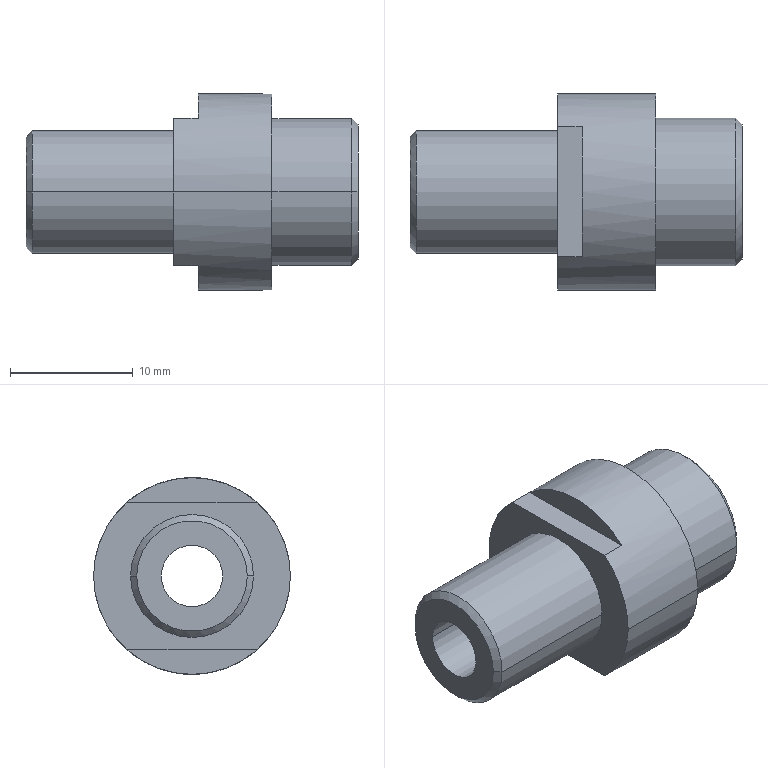Component | SolidWorks | ClampingAssembly-1_A72-1 | 1 solid | 20 faces | box 27 x 16 x 16 mm | volume 2746 mm3 | cylinder 8 | plane 8 | cone 4 | commonest cylinder face diameters 5 x2 10 x2 16 x2 12 x2 | material S45C
build123d program:
from build123d import *
from build123d.topology import SkipClean

# Parameters (mm, degrees)
SKETCH1_R             = 6
BOSS_EXTRUDE1_DEPTH   = 7
SKETCH2_R             = 8
BOSS_EXTRUDE2_DEPTH   = 6
CHAMFER1_SIZE         = 0.5
BOSS_EXTRUDE3_DEPTH   = 2
SKETCH4_R             = 5
BOSS_EXTRUDE4_DEPTH   = 12
M5_TAPPED_HOLE1_D     = 5
M5_TAPPED_HOLE1_DEPTH = 12.4
M5_TAPPED_HOLE1_TIP   = 1.502
M6_TAPPED_HOLE2_D     = 5
M6_TAPPED_HOLE2_DEPTH = 15
M6_TAPPED_HOLE2_TIP   = 1.502
CHAMFER2_SIZE         = 0.5


with BuildPart() as part:
    # Sketch1 → Boss-Extrude1 (new body)
    with BuildSketch(Plane(origin=(0, 0, 0), x_dir=(0, 0, -1), z_dir=(1, 0, 0))):
        Circle(SKETCH1_R)
    extrude(amount=BOSS_EXTRUDE1_DEPTH)

    # Sketch2 → Boss-Extrude2 (add)
    with BuildSketch(Plane.ZY):
        Circle(SKETCH2_R)
    extrude(amount=BOSS_EXTRUDE2_DEPTH)

    # Chamfer1
    chamfer1_edges = [part.edges().sort_by_distance(p)[0] for p in [
        (7, 0, 6),
    ]]
    chamfer(chamfer1_edges, length=CHAMFER1_SIZE)

    # Sketch3 → Boss-Extrude3 (add)
    with SkipClean():  # the faces are left unmerged after this step: merging them gives an invalid solid
        with BuildSketch(Plane.ZY.offset(6)):
            with BuildLine():
                Line((-5.292, 6), (5.292, 6))
                ThreePointArc((5.292, 6), (8, 0), (5.292, -6))
                Line((5.292, -6), (-5.292, -6))
                ThreePointArc((-5.292, -6), (-8, 0), (-5.292, 6))
            make_face()
        extrude(amount=BOSS_EXTRUDE3_DEPTH)

    # Sketch4 → Boss-Extrude4 (add)
    with SkipClean():  # the faces are left unmerged after this step: merging them gives an invalid solid
        with BuildSketch(Plane.ZY.offset(8)):
            Circle(SKETCH4_R)
        extrude(amount=BOSS_EXTRUDE4_DEPTH)

    # M5 Tapped Hole1
    with Locations(Plane(origin=(7, 0, 0), x_dir=(0, 0, -1), z_dir=(1, 0, 0))):
        with Locations((0, 0)):
            Hole(M5_TAPPED_HOLE1_D / 2, depth=M5_TAPPED_HOLE1_DEPTH)
            with Locations((0, 0, -(M5_TAPPED_HOLE1_DEPTH + M5_TAPPED_HOLE1_TIP / 2))):  # 118° drill point
                Cone(0, M5_TAPPED_HOLE1_D / 2, M5_TAPPED_HOLE1_TIP, mode=Mode.SUBTRACT)

    # M6 Tapped Hole2
    with Locations(Plane.ZY.offset(20)):
        with Locations((0, 0)):
            Hole(M6_TAPPED_HOLE2_D / 2, depth=M6_TAPPED_HOLE2_DEPTH)
            with Locations((0, 0, -(M6_TAPPED_HOLE2_DEPTH + M6_TAPPED_HOLE2_TIP / 2))):  # 118° drill point
                Cone(0, M6_TAPPED_HOLE2_D / 2, M6_TAPPED_HOLE2_TIP, mode=Mode.SUBTRACT)

    # Chamfer2
    chamfer2_edges = [part.edges().sort_by_distance(p)[0] for p in [
        (-20, 0, -5),
    ]]
    chamfer(chamfer2_edges, length=CHAMFER2_SIZE)


solid = part.part

# Placed as in the assembly
solid = solid.moved(Location((-29.551, 66.036, -52.5), (90, 0, 0)))
STEP:
#1=CARTESIAN_POINT('',(-1.951,2.777,-2.067));
#2=VERTEX_POINT('',#1);
#3=CARTESIAN_POINT('',(-1.951,2.423,-2.067));
#4=VERTEX_POINT('',#3);
#5=CARTESIAN_POINT('',(-1.951,2.6,-2.067));
#6=DIRECTION('',(-1.,-0.,-0.));
#7=DIRECTION('',(0.,1.,-0.0003333));
#8=AXIS2_PLACEMENT_3D('',#5,#6,#7);
#9=CIRCLE('',#8,0.1772);
#10=EDGE_CURVE('',#2,#4,#9,.T.);
#11=ORIENTED_EDGE('',*,*,#10,.F.);
#12=CARTESIAN_POINT('',(-1.931,2.797,-2.067));
#13=VERTEX_POINT('',#12);
#14=CARTESIAN_POINT('',(-1.951,2.777,-2.067));
#15=DIRECTION('',(0.7071,0.7071,-0.0002357));
#16=VECTOR('',#15,39.37);
#17=LINE('',#14,#16);
#18=EDGE_CURVE('',#2,#13,#17,.T.);
#19=ORIENTED_EDGE('',*,*,#18,.T.);
#20=CARTESIAN_POINT('',(-1.931,2.403,-2.067));
#21=VERTEX_POINT('',#20);
#22=CARTESIAN_POINT('',(-1.931,2.6,-2.067));
#23=DIRECTION('',(1.,0.,0.));
#24=DIRECTION('',(0.,1.,-0.0003333));
#25=AXIS2_PLACEMENT_3D('',#22,#23,#24);
#26=CIRCLE('',#25,0.1969);
#27=EDGE_CURVE('',#21,#13,#26,.T.);
#28=ORIENTED_EDGE('',*,*,#27,.F.);
#29=CARTESIAN_POINT('',(-1.951,2.423,-2.067));
#30=DIRECTION('',(0.7071,-0.7071,0.0002357));
#31=VECTOR('',#30,39.37);
#32=LINE('',#29,#31);
#33=EDGE_CURVE('',#4,#21,#32,.T.);
#34=ORIENTED_EDGE('',*,*,#33,.F.);
#35=EDGE_LOOP('',(#11,#19,#28,#34));
#36=FACE_OUTER_BOUND('',#35,.T.);
#37=CARTESIAN_POINT('',(-1.951,2.6,-2.067));
#38=DIRECTION('',(1.,0.,0.));
#39=DIRECTION('',(0.,-1.,0.0003333));
#40=AXIS2_PLACEMENT_3D('',#37,#38,#39);
#41=CONICAL_SURFACE('',#40,0.1772,0.7854);
#42=ADVANCED_FACE('',(#36),#41,.T.);
#43=CARTESIAN_POINT('',(-1.951,2.501,-2.067));
#44=VERTEX_POINT('',#43);
#45=CARTESIAN_POINT('',(-1.951,2.698,-2.067));
#46=VERTEX_POINT('',#45);
#47=CARTESIAN_POINT('',(-1.951,2.6,-2.067));
#48=DIRECTION('',(-1.,-0.,-0.));
#49=DIRECTION('',(0.,1.,-0.0003333));
#50=AXIS2_PLACEMENT_3D('',#47,#48,#49);
#51=CIRCLE('',#50,0.09843);
#52=EDGE_CURVE('',#44,#46,#51,.T.);
#53=ORIENTED_EDGE('',*,*,#52,.T.);
#54=CARTESIAN_POINT('',(-0.8878,2.698,-2.067));
#55=VERTEX_POINT('',#54);
#56=CARTESIAN_POINT('',(-0.8878,2.698,-2.067));
#57=DIRECTION('',(1.,0.,0.));
#58=VECTOR('',#57,39.37);
#59=LINE('',#56,#58);
#60=EDGE_CURVE('',#46,#55,#59,.T.);
#61=ORIENTED_EDGE('',*,*,#60,.T.);
#62=CARTESIAN_POINT('',(-0.8878,2.501,-2.067));
#63=VERTEX_POINT('',#62);
#64=CARTESIAN_POINT('',(-0.8878,2.6,-2.067));
#65=DIRECTION('',(1.,0.,0.));
#66=DIRECTION('',(0.,-1.,0.0003333));
#67=AXIS2_PLACEMENT_3D('',#64,#65,#66);
#68=CIRCLE('',#67,0.09843);
#69=EDGE_CURVE('',#55,#63,#68,.T.);
#70=ORIENTED_EDGE('',*,*,#69,.T.);
#71=CARTESIAN_POINT('',(-0.8878,2.501,-2.067));
#72=DIRECTION('',(1.,0.,0.));
#73=VECTOR('',#72,39.37);
#74=LINE('',#71,#73);
#75=EDGE_CURVE('',#44,#63,#74,.T.);
#76=ORIENTED_EDGE('',*,*,#75,.F.);
#77=EDGE_LOOP('',(#53,#61,#70,#76));
#78=FACE_OUTER_BOUND('',#77,.T.);
#79=CARTESIAN_POINT('',(-0.8878,2.6,-2.067));
#80=DIRECTION('',(1.,0.,0.));
#81=DIRECTION('',(0.,-1.,0.0003333));
#82=AXIS2_PLACEMENT_3D('',#79,#80,#81);
#83=CYLINDRICAL_SURFACE('',#82,0.09843);
#84=ADVANCED_FACE('',(#78),#83,.F.);
#85=ORIENTED_EDGE('',*,*,#27,.T.);
#86=CARTESIAN_POINT('',(-1.478,2.797,-2.067));
#87=VERTEX_POINT('',#86);
#88=CARTESIAN_POINT('',(-1.951,2.797,-2.067));
#89=DIRECTION('',(1.,0.,0.));
#90=VECTOR('',#89,39.37);
#91=LINE('',#88,#90);
#92=EDGE_CURVE('',#13,#87,#91,.T.);
#93=ORIENTED_EDGE('',*,*,#92,.T.);
#94=CARTESIAN_POINT('',(-1.478,2.403,-2.067));
#95=VERTEX_POINT('',#94);
#96=CARTESIAN_POINT('',(-1.478,2.6,-2.067));
#97=DIRECTION('',(-1.,-0.,-0.));
#98=DIRECTION('',(0.,1.,-0.0003333));
#99=AXIS2_PLACEMENT_3D('',#96,#97,#98);
#100=CIRCLE('',#99,0.1969);
#101=EDGE_CURVE('',#87,#95,#100,.T.);
#102=ORIENTED_EDGE('',*,*,#101,.T.);
#103=CARTESIAN_POINT('',(-1.951,2.403,-2.067));
#104=DIRECTION('',(1.,0.,0.));
#105=VECTOR('',#104,39.37);
#106=LINE('',#103,#105);
#107=EDGE_CURVE('',#21,#95,#106,.T.);
#108=ORIENTED_EDGE('',*,*,#107,.F.);
#109=EDGE_LOOP('',(#85,#93,#102,#108));
#110=FACE_OUTER_BOUND('',#109,.T.);
#111=CARTESIAN_POINT('',(-1.951,2.6,-2.067));
#112=DIRECTION('',(1.,0.,0.));
#113=DIRECTION('',(0.,-1.,0.0003333));
#114=AXIS2_PLACEMENT_3D('',#111,#112,#113);
#115=CYLINDRICAL_SURFACE('',#114,0.1969);
#116=ADVANCED_FACE('',(#110),#115,.T.);
#117=CARTESIAN_POINT('',(-0.8878,2.383,-2.067));
#118=VERTEX_POINT('',#117);
#119=CARTESIAN_POINT('',(-0.8878,2.816,-2.067));
#120=VERTEX_POINT('',#119);
#121=CARTESIAN_POINT('',(-0.8878,2.6,-2.067));
#122=DIRECTION('',(1.,0.,0.));
#123=DIRECTION('',(0.,-1.,0.0003333));
#124=AXIS2_PLACEMENT_3D('',#121,#122,#123);
#125=CIRCLE('',#124,0.2165);
#126=EDGE_CURVE('',#118,#120,#125,.T.);
#127=ORIENTED_EDGE('',*,*,#126,.F.);
#128=CARTESIAN_POINT('',(-0.9075,2.364,-2.067));
#129=VERTEX_POINT('',#128);
#130=CARTESIAN_POINT('',(-0.8878,2.383,-2.067));
#131=DIRECTION('',(-0.7071,-0.7071,0.0002357));
#132=VECTOR('',#131,39.37);
#133=LINE('',#130,#132);
#134=EDGE_CURVE('',#118,#129,#133,.T.);
#135=ORIENTED_EDGE('',*,*,#134,.T.);
#136=CARTESIAN_POINT('',(-0.9075,2.836,-2.067));
#137=VERTEX_POINT('',#136);
#138=CARTESIAN_POINT('',(-0.9075,2.6,-2.067));
#139=DIRECTION('',(-1.,-0.,-0.));
#140=DIRECTION('',(0.,-1.,0.0003333));
#141=AXIS2_PLACEMENT_3D('',#138,#139,#140);
#142=CIRCLE('',#141,0.2362);
#143=EDGE_CURVE('',#137,#129,#142,.T.);
#144=ORIENTED_EDGE('',*,*,#143,.F.);
#145=CARTESIAN_POINT('',(-0.8878,2.816,-2.067));
#146=DIRECTION('',(-0.7071,0.7071,-0.0002357));
#147=VECTOR('',#146,39.37);
#148=LINE('',#145,#147);
#149=EDGE_CURVE('',#120,#137,#148,.T.);
#150=ORIENTED_EDGE('',*,*,#149,.F.);
#151=EDGE_LOOP('',(#127,#135,#144,#150));
#152=FACE_OUTER_BOUND('',#151,.T.);
#153=CARTESIAN_POINT('',(-0.8878,2.6,-2.067));
#154=DIRECTION('',(-1.,-0.,-0.));
#155=DIRECTION('',(0.,1.,-0.0003333));
#156=AXIS2_PLACEMENT_3D('',#153,#154,#155);
#157=CONICAL_SURFACE('',#156,0.2165,0.7854);
#158=ADVANCED_FACE('',(#152),#157,.T.);
#159=CARTESIAN_POINT('',(-1.478,2.915,-2.067));
#160=VERTEX_POINT('',#159);
#161=CARTESIAN_POINT('',(-1.478,2.808,-2.303));
#162=VERTEX_POINT('',#161);
#163=CARTESIAN_POINT('',(-1.478,2.6,-2.067));
#164=DIRECTION('',(-1.,-0.,-0.));
#165=DIRECTION('',(0.,1.,-0.0003333));
#166=AXIS2_PLACEMENT_3D('',#163,#164,#165);
#167=CIRCLE('',#166,0.315);
#168=EDGE_CURVE('',#160,#162,#167,.T.);
#169=ORIENTED_EDGE('',*,*,#168,.F.);
#170=CARTESIAN_POINT('',(-1.163,2.915,-2.067));
#171=VERTEX_POINT('',#170);
#172=CARTESIAN_POINT('',(-1.4,2.915,-2.067));
#173=DIRECTION('',(1.,0.,0.));
#174=VECTOR('',#173,39.37);
#175=LINE('',#172,#174);
#176=EDGE_CURVE('',#160,#171,#175,.T.);
#177=ORIENTED_EDGE('',*,*,#176,.T.);
#178=CARTESIAN_POINT('',(-1.163,2.285,-2.067));
#179=VERTEX_POINT('',#178);
#180=CARTESIAN_POINT('',(-1.163,2.6,-2.067));
#181=DIRECTION('',(-1.,-0.,-0.));
#182=DIRECTION('',(0.,1.,-0.0003333));
#183=AXIS2_PLACEMENT_3D('',#180,#181,#182);
#184=CIRCLE('',#183,0.315);
#185=EDGE_CURVE('',#171,#179,#184,.T.);
#186=ORIENTED_EDGE('',*,*,#185,.T.);
#187=CARTESIAN_POINT('',(-1.478,2.285,-2.067));
#188=VERTEX_POINT('',#187);
#189=CARTESIAN_POINT('',(-1.4,2.285,-2.067));
#190=DIRECTION('',(1.,0.,0.));
#191=VECTOR('',#190,39.37);
#192=LINE('',#189,#191);
#193=EDGE_CURVE('',#188,#179,#192,.T.);
#194=ORIENTED_EDGE('',*,*,#193,.F.);
#195=CARTESIAN_POINT('',(-1.478,2.391,-2.303));
#196=VERTEX_POINT('',#195);
#197=CARTESIAN_POINT('',(-1.478,2.6,-2.067));
#198=DIRECTION('',(-1.,-0.,-0.));
#199=DIRECTION('',(0.,1.,-0.0003333));
#200=AXIS2_PLACEMENT_3D('',#197,#198,#199);
#201=CIRCLE('',#200,0.315);
#202=EDGE_CURVE('',#196,#188,#201,.T.);
#203=ORIENTED_EDGE('',*,*,#202,.F.);
#204=CARTESIAN_POINT('',(-1.4,2.391,-2.303));
#205=VERTEX_POINT('',#204);
#206=CARTESIAN_POINT('',(-1.478,2.391,-2.303));
#207=DIRECTION('',(1.,0.,0.));
#208=VECTOR('',#207,39.37);
#209=LINE('',#206,#208);
#210=EDGE_CURVE('',#196,#205,#209,.T.);
#211=ORIENTED_EDGE('',*,*,#210,.T.);
#212=CARTESIAN_POINT('',(-1.4,2.808,-2.303));
#213=VERTEX_POINT('',#212);
#214=CARTESIAN_POINT('',(-1.4,2.6,-2.067));
#215=DIRECTION('',(-1.,-0.,-0.));
#216=DIRECTION('',(0.,1.,-0.0003333));
#217=AXIS2_PLACEMENT_3D('',#214,#215,#216);
#218=CIRCLE('',#217,0.315);
#219=EDGE_CURVE('',#213,#205,#218,.T.);
#220=ORIENTED_EDGE('',*,*,#219,.F.);
#221=CARTESIAN_POINT('',(-1.478,2.808,-2.303));
#222=DIRECTION('',(1.,0.,0.));
#223=VECTOR('',#222,39.37);
#224=LINE('',#221,#223);
#225=EDGE_CURVE('',#162,#213,#224,.T.);
#226=ORIENTED_EDGE('',*,*,#225,.F.);
#227=EDGE_LOOP('',(#169,#177,#186,#194,#203,#211,#220,#226));
#228=FACE_OUTER_BOUND('',#227,.T.);
#229=CARTESIAN_POINT('',(-1.4,2.6,-2.067));
#230=DIRECTION('',(1.,0.,0.));
#231=DIRECTION('',(0.,-1.,0.0003333));
#232=AXIS2_PLACEMENT_3D('',#229,#230,#231);
#233=CYLINDRICAL_SURFACE('',#232,0.315);
#234=ADVANCED_FACE('',(#228),#233,.T.);
#235=ORIENTED_EDGE('',*,*,#143,.T.);
#236=CARTESIAN_POINT('',(-1.163,2.364,-2.067));
#237=VERTEX_POINT('',#236);
#238=CARTESIAN_POINT('',(-0.8878,2.364,-2.067));
#239=DIRECTION('',(-1.,-0.,-0.));
#240=VECTOR('',#239,39.37);
#241=LINE('',#238,#240);
#242=EDGE_CURVE('',#129,#237,#241,.T.);
#243=ORIENTED_EDGE('',*,*,#242,.T.);
#244=CARTESIAN_POINT('',(-1.163,2.836,-2.067));
#245=VERTEX_POINT('',#244);
#246=CARTESIAN_POINT('',(-1.163,2.6,-2.067));
#247=DIRECTION('',(1.,0.,0.));
#248=DIRECTION('',(0.,-1.,0.0003333));
#249=AXIS2_PLACEMENT_3D('',#246,#247,#248);
#250=CIRCLE('',#249,0.2362);
#251=EDGE_CURVE('',#237,#245,#250,.T.);
#252=ORIENTED_EDGE('',*,*,#251,.T.);
#253=CARTESIAN_POINT('',(-0.8878,2.836,-2.067));
#254=DIRECTION('',(-1.,-0.,-0.));
#255=VECTOR('',#254,39.37);
#256=LINE('',#253,#255);
#257=EDGE_CURVE('',#137,#245,#256,.T.);
#258=ORIENTED_EDGE('',*,*,#257,.F.);
#259=EDGE_LOOP('',(#235,#243,#252,#258));
#260=FACE_OUTER_BOUND('',#259,.T.);
#261=CARTESIAN_POINT('',(-0.8878,2.6,-2.067));
#262=DIRECTION('',(-1.,-0.,-0.));
#263=DIRECTION('',(0.,1.,-0.0003333));
#264=AXIS2_PLACEMENT_3D('',#261,#262,#263);
#265=CYLINDRICAL_SURFACE('',#264,0.2362);
#266=ADVANCED_FACE('',(#260),#265,.T.);
#267=CARTESIAN_POINT('',(-1.4,2.391,-2.303));
#268=DIRECTION('',(0.,-1.,0.0003333));
#269=VECTOR('',#268,39.37);
#270=LINE('',#267,#269);
#271=EDGE_CURVE('',#213,#205,#270,.T.);
#272=ORIENTED_EDGE('',*,*,#271,.F.);
#273=ORIENTED_EDGE('',*,*,#219,.T.);
#274=EDGE_LOOP('',(#272,#273));
#275=FACE_OUTER_BOUND('',#274,.T.);
#276=CARTESIAN_POINT('',(-1.4,2.6,-2.067));
#277=DIRECTION('',(-1.,-0.,-0.));
#278=DIRECTION('',(-0.,1.,-0.0003333));
#279=AXIS2_PLACEMENT_3D('',#276,#277,#278);
#280=PLANE('',#279);
#281=ADVANCED_FACE('',(#275),#280,.T.);
#282=ORIENTED_EDGE('',*,*,#242,.F.);
#283=CARTESIAN_POINT('',(-0.9075,2.6,-2.067));
#284=DIRECTION('',(-1.,-0.,-0.));
#285=DIRECTION('',(0.,-1.,0.0003333));
#286=AXIS2_PLACEMENT_3D('',#283,#284,#285);
#287=CIRCLE('',#286,0.2362);
#288=EDGE_CURVE('',#129,#137,#287,.T.);
#289=ORIENTED_EDGE('',*,*,#288,.T.);
#290=ORIENTED_EDGE('',*,*,#257,.T.);
#291=CARTESIAN_POINT('',(-1.163,2.6,-2.067));
#292=DIRECTION('',(1.,0.,0.));
#293=DIRECTION('',(0.,-1.,0.0003333));
#294=AXIS2_PLACEMENT_3D('',#291,#292,#293);
#295=CIRCLE('',#294,0.2362);
#296=EDGE_CURVE('',#245,#237,#295,.T.);
#297=ORIENTED_EDGE('',*,*,#296,.T.);
#298=EDGE_LOOP('',(#282,#289,#290,#297));
#299=FACE_OUTER_BOUND('',#298,.T.);
#300=CARTESIAN_POINT('',(-0.8878,2.6,-2.067));
#301=DIRECTION('',(-1.,-0.,-0.));
#302=DIRECTION('',(0.,1.,-0.0003333));
#303=AXIS2_PLACEMENT_3D('',#300,#301,#302);
#304=CYLINDRICAL_SURFACE('',#303,0.2362);
#305=ADVANCED_FACE('',(#299),#304,.T.);
#306=CARTESIAN_POINT('',(-0.8878,2.6,-2.067));
#307=DIRECTION('',(1.,0.,0.));
#308=DIRECTION('',(0.,-1.,0.0003333));
#309=AXIS2_PLACEMENT_3D('',#306,#307,#308);
#310=CIRCLE('',#309,0.09843);
#311=EDGE_CURVE('',#63,#55,#310,.T.);
#312=ORIENTED_EDGE('',*,*,#311,.F.);
#313=ORIENTED_EDGE('',*,*,#69,.F.);
#314=EDGE_LOOP('',(#312,#313));
#315=FACE_BOUND('',#314,.T.);
#316=CARTESIAN_POINT('',(-0.8878,2.6,-2.067));
#317=DIRECTION('',(1.,0.,0.));
#318=DIRECTION('',(0.,-1.,0.0003333));
#319=AXIS2_PLACEMENT_3D('',#316,#317,#318);
#320=CIRCLE('',#319,0.2165);
#321=EDGE_CURVE('',#120,#118,#320,.T.);
#322=ORIENTED_EDGE('',*,*,#321,.T.);
#323=ORIENTED_EDGE('',*,*,#126,.T.);
#324=EDGE_LOOP('',(#322,#323));
#325=FACE_OUTER_BOUND('',#324,.T.);
#326=CARTESIAN_POINT('',(-0.8878,2.6,-2.067));
#327=DIRECTION('',(1.,0.,0.));
#328=DIRECTION('',(0.,-1.,0.0003333));
#329=AXIS2_PLACEMENT_3D('',#326,#327,#328);
#330=PLANE('',#329);
#331=ADVANCED_FACE('',(#315,#325),#330,.T.);
#332=ORIENTED_EDGE('',*,*,#176,.F.);
#333=CARTESIAN_POINT('',(-1.478,2.808,-1.831));
#334=VERTEX_POINT('',#333);
#335=CARTESIAN_POINT('',(-1.478,2.6,-2.067));
#336=DIRECTION('',(-1.,-0.,-0.));
#337=DIRECTION('',(0.,1.,-0.0003333));
#338=AXIS2_PLACEMENT_3D('',#335,#336,#337);
#339=CIRCLE('',#338,0.315);
#340=EDGE_CURVE('',#334,#160,#339,.T.);
#341=ORIENTED_EDGE('',*,*,#340,.F.);
#342=CARTESIAN_POINT('',(-1.4,2.808,-1.831));
#343=VERTEX_POINT('',#342);
#344=CARTESIAN_POINT('',(-1.478,2.808,-1.831));
#345=DIRECTION('',(1.,0.,0.));
#346=VECTOR('',#345,39.37);
#347=LINE('',#344,#346);
#348=EDGE_CURVE('',#334,#343,#347,.T.);
#349=ORIENTED_EDGE('',*,*,#348,.T.);
#350=CARTESIAN_POINT('',(-1.4,2.392,-1.831));
#351=VERTEX_POINT('',#350);
#352=CARTESIAN_POINT('',(-1.4,2.6,-2.067));
#353=DIRECTION('',(-1.,-0.,-0.));
#354=DIRECTION('',(0.,1.,-0.0003333));
#355=AXIS2_PLACEMENT_3D('',#352,#353,#354);
#356=CIRCLE('',#355,0.315);
#357=EDGE_CURVE('',#351,#343,#356,.T.);
#358=ORIENTED_EDGE('',*,*,#357,.F.);
#359=CARTESIAN_POINT('',(-1.478,2.392,-1.831));
#360=VERTEX_POINT('',#359);
#361=CARTESIAN_POINT('',(-1.478,2.392,-1.831));
#362=DIRECTION('',(1.,0.,0.));
#363=VECTOR('',#362,39.37);
#364=LINE('',#361,#363);
#365=EDGE_CURVE('',#360,#351,#364,.T.);
#366=ORIENTED_EDGE('',*,*,#365,.F.);
#367=CARTESIAN_POINT('',(-1.478,2.6,-2.067));
#368=DIRECTION('',(-1.,-0.,-0.));
#369=DIRECTION('',(0.,1.,-0.0003333));
#370=AXIS2_PLACEMENT_3D('',#367,#368,#369);
#371=CIRCLE('',#370,0.315);
#372=EDGE_CURVE('',#188,#360,#371,.T.);
#373=ORIENTED_EDGE('',*,*,#372,.F.);
#374=ORIENTED_EDGE('',*,*,#193,.T.);
#375=CARTESIAN_POINT('',(-1.163,2.6,-2.067));
#376=DIRECTION('',(-1.,-0.,-0.));
#377=DIRECTION('',(0.,1.,-0.0003333));
#378=AXIS2_PLACEMENT_3D('',#375,#376,#377);
#379=CIRCLE('',#378,0.315);
#380=EDGE_CURVE('',#179,#171,#379,.T.);
#381=ORIENTED_EDGE('',*,*,#380,.T.);
#382=EDGE_LOOP('',(#332,#341,#349,#358,#366,#373,#374,#381));
#383=FACE_OUTER_BOUND('',#382,.T.);
#384=CARTESIAN_POINT('',(-1.4,2.6,-2.067));
#385=DIRECTION('',(1.,0.,0.));
#386=DIRECTION('',(0.,-1.,0.0003333));
#387=AXIS2_PLACEMENT_3D('',#384,#385,#386);
#388=CYLINDRICAL_SURFACE('',#387,0.315);
#389=ADVANCED_FACE('',(#383),#388,.T.);
#390=CARTESIAN_POINT('',(-1.4,2.808,-1.831));
#391=DIRECTION('',(-0.,1.,-0.0003333));
#392=VECTOR('',#391,39.37);
#393=LINE('',#390,#392);
#394=EDGE_CURVE('',#351,#343,#393,.T.);
#395=ORIENTED_EDGE('',*,*,#394,.F.);
#396=ORIENTED_EDGE('',*,*,#357,.T.);
#397=EDGE_LOOP('',(#395,#396));
#398=FACE_OUTER_BOUND('',#397,.T.);
#399=CARTESIAN_POINT('',(-1.4,2.6,-2.067));
#400=DIRECTION('',(-1.,-0.,-0.));
#401=DIRECTION('',(-0.,1.,-0.0003333));
#402=AXIS2_PLACEMENT_3D('',#399,#400,#401);
#403=PLANE('',#402);
#404=ADVANCED_FACE('',(#398),#403,.T.);
#405=ORIENTED_EDGE('',*,*,#296,.F.);
#406=ORIENTED_EDGE('',*,*,#251,.F.);
#407=EDGE_LOOP('',(#405,#406));
#408=FACE_BOUND('',#407,.T.);
#409=ORIENTED_EDGE('',*,*,#380,.F.);
#410=ORIENTED_EDGE('',*,*,#185,.F.);
#411=EDGE_LOOP('',(#409,#410));
#412=FACE_OUTER_BOUND('',#411,.T.);
#413=CARTESIAN_POINT('',(-1.163,2.6,-2.067));
#414=DIRECTION('',(-1.,-0.,-0.));
#415=DIRECTION('',(-0.,1.,-0.0003333));
#416=AXIS2_PLACEMENT_3D('',#413,#414,#415);
#417=PLANE('',#416);
#418=ADVANCED_FACE('',(#408,#412),#417,.F.);
#419=ORIENTED_EDGE('',*,*,#134,.F.);
#420=ORIENTED_EDGE('',*,*,#321,.F.);
#421=ORIENTED_EDGE('',*,*,#149,.T.);
#422=ORIENTED_EDGE('',*,*,#288,.F.);
#423=EDGE_LOOP('',(#419,#420,#421,#422));
#424=FACE_OUTER_BOUND('',#423,.T.);
#425=CARTESIAN_POINT('',(-0.8878,2.6,-2.067));
#426=DIRECTION('',(-1.,-0.,-0.));
#427=DIRECTION('',(0.,1.,-0.0003333));
#428=AXIS2_PLACEMENT_3D('',#425,#426,#427);
#429=CONICAL_SURFACE('',#428,0.2165,0.7854);
#430=ADVANCED_FACE('',(#424),#429,.T.);
#431=ORIENTED_EDGE('',*,*,#394,.T.);
#432=ORIENTED_EDGE('',*,*,#348,.F.);
#433=CARTESIAN_POINT('',(-1.478,2.808,-1.831));
#434=DIRECTION('',(-0.,1.,-0.0003333));
#435=VECTOR('',#434,39.37);
#436=LINE('',#433,#435);
#437=EDGE_CURVE('',#360,#334,#436,.T.);
#438=ORIENTED_EDGE('',*,*,#437,.F.);
#439=ORIENTED_EDGE('',*,*,#365,.T.);
#440=EDGE_LOOP('',(#431,#432,#438,#439));
#441=FACE_OUTER_BOUND('',#440,.T.);
#442=CARTESIAN_POINT('',(-1.478,2.808,-1.831));
#443=DIRECTION('',(0.,-0.0003333,-1.));
#444=DIRECTION('',(-0.,1.,-0.0003333));
#445=AXIS2_PLACEMENT_3D('',#442,#443,#444);
#446=PLANE('',#445);
#447=ADVANCED_FACE('',(#441),#446,.F.);
#448=ORIENTED_EDGE('',*,*,#271,.T.);
#449=ORIENTED_EDGE('',*,*,#210,.F.);
#450=CARTESIAN_POINT('',(-1.478,2.391,-2.303));
#451=DIRECTION('',(0.,-1.,0.0003333));
#452=VECTOR('',#451,39.37);
#453=LINE('',#450,#452);
#454=EDGE_CURVE('',#162,#196,#453,.T.);
#455=ORIENTED_EDGE('',*,*,#454,.F.);
#456=ORIENTED_EDGE('',*,*,#225,.T.);
#457=EDGE_LOOP('',(#448,#449,#455,#456));
#458=FACE_OUTER_BOUND('',#457,.T.);
#459=CARTESIAN_POINT('',(-1.478,2.391,-2.303));
#460=DIRECTION('',(-0.,0.0003333,1.));
#461=DIRECTION('',(0.,-1.,0.0003333));
#462=AXIS2_PLACEMENT_3D('',#459,#460,#461);
#463=PLANE('',#462);
#464=ADVANCED_FACE('',(#458),#463,.F.);
#465=CARTESIAN_POINT('',(-1.478,2.6,-2.067));
#466=DIRECTION('',(-1.,-0.,-0.));
#467=DIRECTION('',(0.,1.,-0.0003333));
#468=AXIS2_PLACEMENT_3D('',#465,#466,#467);
#469=CIRCLE('',#468,0.1969);
#470=EDGE_CURVE('',#95,#87,#469,.T.);
#471=ORIENTED_EDGE('',*,*,#470,.F.);
#472=ORIENTED_EDGE('',*,*,#101,.F.);
#473=EDGE_LOOP('',(#471,#472));
#474=FACE_BOUND('',#473,.T.);
#475=ORIENTED_EDGE('',*,*,#202,.T.);
#476=ORIENTED_EDGE('',*,*,#372,.T.);
#477=ORIENTED_EDGE('',*,*,#437,.T.);
#478=ORIENTED_EDGE('',*,*,#340,.T.);
#479=ORIENTED_EDGE('',*,*,#168,.T.);
#480=ORIENTED_EDGE('',*,*,#454,.T.);
#481=EDGE_LOOP('',(#475,#476,#477,#478,#479,#480));
#482=FACE_OUTER_BOUND('',#481,.T.);
#483=CARTESIAN_POINT('',(-1.478,2.6,-2.067));
#484=DIRECTION('',(-1.,-0.,-0.));
#485=DIRECTION('',(-0.,1.,-0.0003333));
#486=AXIS2_PLACEMENT_3D('',#483,#484,#485);
#487=PLANE('',#486);
#488=ADVANCED_FACE('',(#474,#482),#487,.T.);
#489=ORIENTED_EDGE('',*,*,#92,.F.);
#490=CARTESIAN_POINT('',(-1.931,2.6,-2.067));
#491=DIRECTION('',(1.,0.,0.));
#492=DIRECTION('',(0.,1.,-0.0003333));
#493=AXIS2_PLACEMENT_3D('',#490,#491,#492);
#494=CIRCLE('',#493,0.1969);
#495=EDGE_CURVE('',#13,#21,#494,.T.);
#496=ORIENTED_EDGE('',*,*,#495,.T.);
#497=ORIENTED_EDGE('',*,*,#107,.T.);
#498=ORIENTED_EDGE('',*,*,#470,.T.);
#499=EDGE_LOOP('',(#489,#496,#497,#498));
#500=FACE_OUTER_BOUND('',#499,.T.);
#501=CARTESIAN_POINT('',(-1.951,2.6,-2.067));
#502=DIRECTION('',(1.,0.,0.));
#503=DIRECTION('',(0.,-1.,0.0003333));
#504=AXIS2_PLACEMENT_3D('',#501,#502,#503);
#505=CYLINDRICAL_SURFACE('',#504,0.1969);
#506=ADVANCED_FACE('',(#500),#505,.T.);
#507=CARTESIAN_POINT('',(-1.951,2.6,-2.067));
#508=DIRECTION('',(-1.,-0.,-0.));
#509=DIRECTION('',(0.,1.,-0.0003333));
#510=AXIS2_PLACEMENT_3D('',#507,#508,#509);
#511=CIRCLE('',#510,0.1772);
#512=EDGE_CURVE('',#4,#2,#511,.T.);
#513=ORIENTED_EDGE('',*,*,#512,.T.);
#514=ORIENTED_EDGE('',*,*,#10,.T.);
#515=EDGE_LOOP('',(#513,#514));
#516=FACE_OUTER_BOUND('',#515,.T.);
#517=ORIENTED_EDGE('',*,*,#52,.F.);
#518=CARTESIAN_POINT('',(-1.951,2.6,-2.067));
#519=DIRECTION('',(-1.,-0.,-0.));
#520=DIRECTION('',(0.,1.,-0.0003333));
#521=AXIS2_PLACEMENT_3D('',#518,#519,#520);
#522=CIRCLE('',#521,0.09843);
#523=EDGE_CURVE('',#46,#44,#522,.T.);
#524=ORIENTED_EDGE('',*,*,#523,.F.);
#525=EDGE_LOOP('',(#517,#524));
#526=FACE_BOUND('',#525,.T.);
#527=CARTESIAN_POINT('',(-1.951,2.6,-2.067));
#528=DIRECTION('',(-1.,-0.,-0.));
#529=DIRECTION('',(-0.,1.,-0.0003333));
#530=AXIS2_PLACEMENT_3D('',#527,#528,#529);
#531=PLANE('',#530);
#532=ADVANCED_FACE('',(#516,#526),#531,.T.);
#533=ORIENTED_EDGE('',*,*,#60,.F.);
#534=ORIENTED_EDGE('',*,*,#523,.T.);
#535=ORIENTED_EDGE('',*,*,#75,.T.);
#536=ORIENTED_EDGE('',*,*,#311,.T.);
#537=EDGE_LOOP('',(#533,#534,#535,#536));
#538=FACE_OUTER_BOUND('',#537,.T.);
#539=CARTESIAN_POINT('',(-0.8878,2.6,-2.067));
#540=DIRECTION('',(1.,0.,0.));
#541=DIRECTION('',(0.,-1.,0.0003333));
#542=AXIS2_PLACEMENT_3D('',#539,#540,#541);
#543=CYLINDRICAL_SURFACE('',#542,0.09843);
#544=ADVANCED_FACE('',(#538),#543,.F.);
#545=ORIENTED_EDGE('',*,*,#18,.F.);
#546=ORIENTED_EDGE('',*,*,#512,.F.);
#547=ORIENTED_EDGE('',*,*,#33,.T.);
#548=ORIENTED_EDGE('',*,*,#495,.F.);
#549=EDGE_LOOP('',(#545,#546,#547,#548));
#550=FACE_OUTER_BOUND('',#549,.T.);
#551=CARTESIAN_POINT('',(-1.951,2.6,-2.067));
#552=DIRECTION('',(1.,0.,0.));
#553=DIRECTION('',(0.,-1.,0.0003333));
#554=AXIS2_PLACEMENT_3D('',#551,#552,#553);
#555=CONICAL_SURFACE('',#554,0.1772,0.7854);
#556=ADVANCED_FACE('',(#550),#555,.T.);
#557=CLOSED_SHELL('',(#42,#84,#116,#158,#234,#266,#281,#305,#331,#389,#404,#418,#430,#447,#464,#488,#506,#532,#544,#556));
#558=MANIFOLD_SOLID_BREP('',#557);
#559=CARTESIAN_POINT('',(0.,0.,0.));
#560=DIRECTION('',(0.,0.,1.));
#561=DIRECTION('',(1.,0.,0.));
#562=AXIS2_PLACEMENT_3D('',#559,#560,#561);
#563=(LENGTH_UNIT()NAMED_UNIT(*)SI_UNIT($,.METRE.));
#564=LENGTH_MEASURE_WITH_UNIT(LENGTH_MEASURE(0.0254),#563);
#565=DIMENSIONAL_EXPONENTS(1.,0.,0.,0.,0.,0.,0.);
#566=(CONVERSION_BASED_UNIT('',#564)LENGTH_UNIT()NAMED_UNIT(#565));
#567=UNCERTAINTY_MEASURE_WITH_UNIT(LENGTH_MEASURE(0.00001),#566,'','');
#568=(NAMED_UNIT(*)PLANE_ANGLE_UNIT()SI_UNIT($,.RADIAN.));
#569=(NAMED_UNIT(*)SI_UNIT($,.STERADIAN.)SOLID_ANGLE_UNIT());
#570=(GEOMETRIC_REPRESENTATION_CONTEXT(3)GLOBAL_UNCERTAINTY_ASSIGNED_CONTEXT((#567))GLOBAL_UNIT_ASSIGNED_CONTEXT((#566,#568,#569))REPRESENTATION_CONTEXT('',''));
#571=ADVANCED_BREP_SHAPE_REPRESENTATION('',(#558,#562),#570);
#572=COLOUR_RGB('',0.7922,0.8196,0.9333);
#573=FILL_AREA_STYLE_COLOUR('',#572);
#574=FILL_AREA_STYLE('',(#573));
#575=SURFACE_STYLE_FILL_AREA(#574);
#576=SURFACE_SIDE_STYLE('',(#575));
#577=SURFACE_STYLE_USAGE(.BOTH.,#576);
#578=PRESENTATION_STYLE_ASSIGNMENT((#577));
#579=STYLED_ITEM('',(#578),#558);
#580=(LENGTH_UNIT()NAMED_UNIT(*)SI_UNIT($,.METRE.));
#581=LENGTH_MEASURE_WITH_UNIT(LENGTH_MEASURE(0.0254),#580);
#582=DIMENSIONAL_EXPONENTS(1.,0.,0.,0.,0.,0.,0.);
#583=(CONVERSION_BASED_UNIT('',#581)LENGTH_UNIT()NAMED_UNIT(#582));
#584=UNCERTAINTY_MEASURE_WITH_UNIT(LENGTH_MEASURE(0.00001),#583,'','');
#585=(NAMED_UNIT(*)PLANE_ANGLE_UNIT()SI_UNIT($,.RADIAN.));
#586=(NAMED_UNIT(*)SI_UNIT($,.STERADIAN.)SOLID_ANGLE_UNIT());
#587=(GEOMETRIC_REPRESENTATION_CONTEXT(3)GLOBAL_UNCERTAINTY_ASSIGNED_CONTEXT((#584))GLOBAL_UNIT_ASSIGNED_CONTEXT((#583,#585,#586))REPRESENTATION_CONTEXT('',''));
#588=MECHANICAL_DESIGN_GEOMETRIC_PRESENTATION_REPRESENTATION('',(#579),#587);
#589=PRESENTATION_LAYER_ASSIGNMENT('','',(#579));